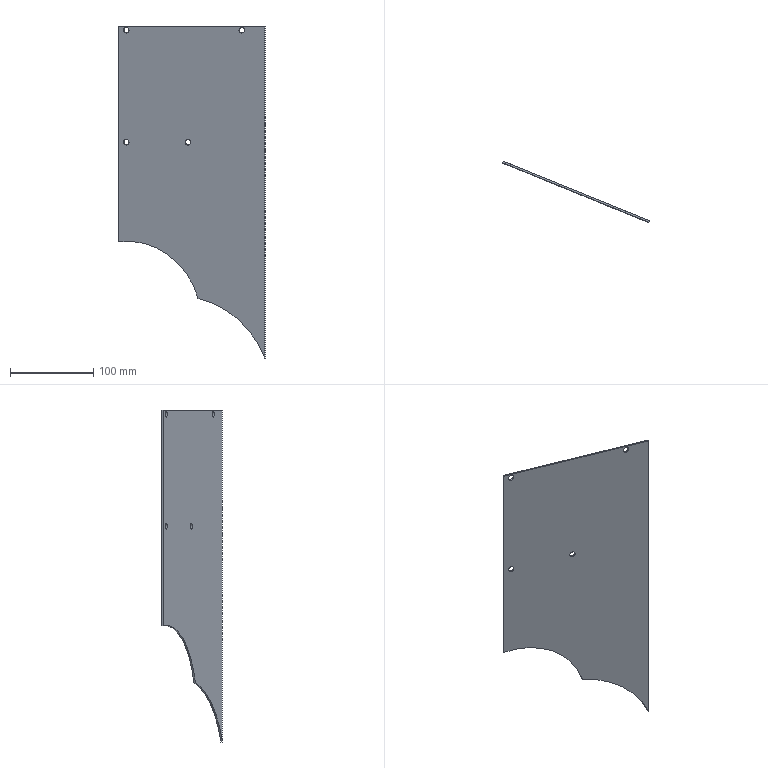Component | SolidWorks | InnerWing-1 | 1 solid | 15 faces | box 176.73 x 73.49 x 400 mm | volume 117704 mm3 | cylinder 10 | plane 5 | commonest cylinder face diameters 7 x8 244.108 x1 192.797 x1
build123d program:
from build123d import *

# Parameters (mm, degrees)
SKETCH1_W           = 190
SKETCH1_H           = 400
BOSS_EXTRUDE1_DEPTH = 2
SKETCH2_R           = 3.5
CUT_EXTRUDE1_DEPTH  = 2
CUT_EXTRUDE2_DEPTH  = 2


with BuildPart() as part:
    # Sketch1 → Boss-Extrude1 (new body)
    with BuildSketch(Plane.XY):
        with Locations((-110.229, 190)):
            Rectangle(SKETCH1_W, SKETCH1_H)
    extrude(amount=BOSS_EXTRUDE1_DEPTH)

    # Sketch2 → Cut-Extrude1 (cut)
    with BuildSketch(Plane.XY.offset(2)):
        with Locations((-195.229, -5)):
            Circle(SKETCH2_R)
        with Locations((-195.229, 130)):
            Circle(SKETCH2_R)
        with Locations((-115.229, 130)):
            Circle(SKETCH2_R)
        with Locations((-45.229, -5)):
            Circle(SKETCH2_R)
    extrude(amount=-CUT_EXTRUDE1_DEPTH, mode=Mode.SUBTRACT)

    # Sketch3 → Cut-Extrude2 (cut)
    with BuildSketch(Plane.XY.offset(2)):
        with BuildLine():
            Line((-205.229, 390), (-205.229, 250))
            ThreePointArc((-205.229, 250), (-141.251, 265.353), (-102.024, 318.174))
            ThreePointArc((-102.024, 318.174), (-49.844, 343.474), (-15.229, 390))
            Line((-15.229, 390), (-205.229, 390))
        make_face()
    extrude(amount=-CUT_EXTRUDE2_DEPTH, mode=Mode.SUBTRACT)


solid = part.part

# Placed as in the assembly
solid = solid.moved(Location((-18.038, -26.671, 107.182), (-90, 22.15, 0)))
STEP:
#1=COLOUR_RGB('',0.7922,0.8196,0.9333);
#2=FILL_AREA_STYLE_COLOUR('',#1);
#3=FILL_AREA_STYLE('',(#2));
#4=SURFACE_STYLE_FILL_AREA(#3);
#5=SURFACE_SIDE_STYLE('',(#4));
#6=SURFACE_STYLE_USAGE(.BOTH.,#5);
#7=PRESENTATION_STYLE_ASSIGNMENT((#6));
#8=CARTESIAN_POINT('',(-2.487,-0.3267,4.417));
#9=VERTEX_POINT('',#8);
#10=CARTESIAN_POINT('',(-2.232,-0.4306,4.417));
#11=VERTEX_POINT('',#10);
#12=CARTESIAN_POINT('',(-2.359,-0.3787,4.417));
#13=DIRECTION('',(0.377,0.9262,-0.));
#14=DIRECTION('',(0.9262,-0.377,0.));
#15=AXIS2_PLACEMENT_3D('',#12,#13,#14);
#16=CIRCLE('',#15,0.1378);
#17=EDGE_CURVE('',#9,#11,#16,.T.);
#18=ORIENTED_EDGE('',*,*,#17,.F.);
#19=CARTESIAN_POINT('',(-2.457,-0.2538,4.417));
#20=VERTEX_POINT('',#19);
#21=CARTESIAN_POINT('',(-2.487,-0.3267,4.417));
#22=DIRECTION('',(0.377,0.9262,-0.));
#23=VECTOR('',#22,39.37);
#24=LINE('',#21,#23);
#25=EDGE_CURVE('',#9,#20,#24,.T.);
#26=ORIENTED_EDGE('',*,*,#25,.T.);
#27=CARTESIAN_POINT('',(-2.202,-0.3577,4.417));
#28=VERTEX_POINT('',#27);
#29=CARTESIAN_POINT('',(-2.33,-0.3057,4.417));
#30=DIRECTION('',(0.377,0.9262,-0.));
#31=DIRECTION('',(0.9262,-0.377,0.));
#32=AXIS2_PLACEMENT_3D('',#29,#30,#31);
#33=CIRCLE('',#32,0.1378);
#34=EDGE_CURVE('',#20,#28,#33,.T.);
#35=ORIENTED_EDGE('',*,*,#34,.T.);
#36=CARTESIAN_POINT('',(-2.232,-0.4306,4.417));
#37=DIRECTION('',(0.377,0.9262,-0.));
#38=VECTOR('',#37,39.37);
#39=LINE('',#36,#38);
#40=EDGE_CURVE('',#11,#28,#39,.T.);
#41=ORIENTED_EDGE('',*,*,#40,.F.);
#42=EDGE_LOOP('',(#18,#26,#35,#41));
#43=FACE_OUTER_BOUND('',#42,.T.);
#44=CARTESIAN_POINT('',(-2.359,-0.3787,4.417));
#45=DIRECTION('',(0.377,0.9262,-0.));
#46=DIRECTION('',(0.9262,-0.377,0.));
#47=AXIS2_PLACEMENT_3D('',#44,#45,#46);
#48=CYLINDRICAL_SURFACE('',#47,0.1378);
#49=ADVANCED_FACE('',(#43),#48,.F.);
#50=CARTESIAN_POINT('',(-5.04,0.7124,-0.8983));
#51=VERTEX_POINT('',#50);
#52=CARTESIAN_POINT('',(-4.784,0.6084,-0.8983));
#53=VERTEX_POINT('',#52);
#54=CARTESIAN_POINT('',(-4.912,0.6604,-0.8983));
#55=DIRECTION('',(0.377,0.9262,-0.));
#56=DIRECTION('',(0.9262,-0.377,0.));
#57=AXIS2_PLACEMENT_3D('',#54,#55,#56);
#58=CIRCLE('',#57,0.1378);
#59=EDGE_CURVE('',#51,#53,#58,.T.);
#60=ORIENTED_EDGE('',*,*,#59,.F.);
#61=CARTESIAN_POINT('',(-5.01,0.7853,-0.8983));
#62=VERTEX_POINT('',#61);
#63=CARTESIAN_POINT('',(-5.04,0.7124,-0.8983));
#64=DIRECTION('',(0.377,0.9262,-0.));
#65=VECTOR('',#64,39.37);
#66=LINE('',#63,#65);
#67=EDGE_CURVE('',#51,#62,#66,.T.);
#68=ORIENTED_EDGE('',*,*,#67,.T.);
#69=CARTESIAN_POINT('',(-4.755,0.6814,-0.8983));
#70=VERTEX_POINT('',#69);
#71=CARTESIAN_POINT('',(-4.882,0.7333,-0.8983));
#72=DIRECTION('',(0.377,0.9262,-0.));
#73=DIRECTION('',(0.9262,-0.377,0.));
#74=AXIS2_PLACEMENT_3D('',#71,#72,#73);
#75=CIRCLE('',#74,0.1378);
#76=EDGE_CURVE('',#62,#70,#75,.T.);
#77=ORIENTED_EDGE('',*,*,#76,.T.);
#78=CARTESIAN_POINT('',(-4.784,0.6084,-0.8983));
#79=DIRECTION('',(0.377,0.9262,-0.));
#80=VECTOR('',#79,39.37);
#81=LINE('',#78,#80);
#82=EDGE_CURVE('',#53,#70,#81,.T.);
#83=ORIENTED_EDGE('',*,*,#82,.F.);
#84=EDGE_LOOP('',(#60,#68,#77,#83));
#85=FACE_OUTER_BOUND('',#84,.T.);
#86=CARTESIAN_POINT('',(-4.912,0.6604,-0.8983));
#87=DIRECTION('',(0.377,0.9262,-0.));
#88=DIRECTION('',(0.9262,-0.377,0.));
#89=AXIS2_PLACEMENT_3D('',#86,#87,#88);
#90=CYLINDRICAL_SURFACE('',#89,0.1378);
#91=ADVANCED_FACE('',(#85),#90,.F.);
#92=CARTESIAN_POINT('',(-7.957,1.9,-0.8983));
#93=VERTEX_POINT('',#92);
#94=CARTESIAN_POINT('',(-7.701,1.796,-0.8983));
#95=VERTEX_POINT('',#94);
#96=CARTESIAN_POINT('',(-7.829,1.848,-0.8983));
#97=DIRECTION('',(0.377,0.9262,-0.));
#98=DIRECTION('',(0.9262,-0.377,0.));
#99=AXIS2_PLACEMENT_3D('',#96,#97,#98);
#100=CIRCLE('',#99,0.1378);
#101=EDGE_CURVE('',#93,#95,#100,.T.);
#102=ORIENTED_EDGE('',*,*,#101,.F.);
#103=CARTESIAN_POINT('',(-7.927,1.973,-0.8983));
#104=VERTEX_POINT('',#103);
#105=CARTESIAN_POINT('',(-7.957,1.9,-0.8983));
#106=DIRECTION('',(0.377,0.9262,-0.));
#107=VECTOR('',#106,39.37);
#108=LINE('',#105,#107);
#109=EDGE_CURVE('',#93,#104,#108,.T.);
#110=ORIENTED_EDGE('',*,*,#109,.T.);
#111=CARTESIAN_POINT('',(-7.672,1.869,-0.8983));
#112=VERTEX_POINT('',#111);
#113=CARTESIAN_POINT('',(-7.799,1.921,-0.8983));
#114=DIRECTION('',(0.377,0.9262,-0.));
#115=DIRECTION('',(0.9262,-0.377,0.));
#116=AXIS2_PLACEMENT_3D('',#113,#114,#115);
#117=CIRCLE('',#116,0.1378);
#118=EDGE_CURVE('',#104,#112,#117,.T.);
#119=ORIENTED_EDGE('',*,*,#118,.T.);
#120=CARTESIAN_POINT('',(-7.701,1.796,-0.8983));
#121=DIRECTION('',(0.377,0.9262,-0.));
#122=VECTOR('',#121,39.37);
#123=LINE('',#120,#122);
#124=EDGE_CURVE('',#95,#112,#123,.T.);
#125=ORIENTED_EDGE('',*,*,#124,.F.);
#126=EDGE_LOOP('',(#102,#110,#119,#125));
#127=FACE_OUTER_BOUND('',#126,.T.);
#128=CARTESIAN_POINT('',(-7.829,1.848,-0.8983));
#129=DIRECTION('',(0.377,0.9262,-0.));
#130=DIRECTION('',(0.9262,-0.377,0.));
#131=AXIS2_PLACEMENT_3D('',#128,#129,#130);
#132=CYLINDRICAL_SURFACE('',#131,0.1378);
#133=ADVANCED_FACE('',(#127),#132,.F.);
#134=CARTESIAN_POINT('',(-7.957,1.9,4.417));
#135=VERTEX_POINT('',#134);
#136=CARTESIAN_POINT('',(-7.701,1.796,4.417));
#137=VERTEX_POINT('',#136);
#138=CARTESIAN_POINT('',(-7.829,1.848,4.417));
#139=DIRECTION('',(0.377,0.9262,-0.));
#140=DIRECTION('',(0.9262,-0.377,0.));
#141=AXIS2_PLACEMENT_3D('',#138,#139,#140);
#142=CIRCLE('',#141,0.1378);
#143=EDGE_CURVE('',#135,#137,#142,.T.);
#144=ORIENTED_EDGE('',*,*,#143,.F.);
#145=CARTESIAN_POINT('',(-7.927,1.973,4.417));
#146=VERTEX_POINT('',#145);
#147=CARTESIAN_POINT('',(-7.957,1.9,4.417));
#148=DIRECTION('',(0.377,0.9262,-0.));
#149=VECTOR('',#148,39.37);
#150=LINE('',#147,#149);
#151=EDGE_CURVE('',#135,#146,#150,.T.);
#152=ORIENTED_EDGE('',*,*,#151,.T.);
#153=CARTESIAN_POINT('',(-7.672,1.869,4.417));
#154=VERTEX_POINT('',#153);
#155=CARTESIAN_POINT('',(-7.799,1.921,4.417));
#156=DIRECTION('',(0.377,0.9262,-0.));
#157=DIRECTION('',(0.9262,-0.377,0.));
#158=AXIS2_PLACEMENT_3D('',#155,#156,#157);
#159=CIRCLE('',#158,0.1378);
#160=EDGE_CURVE('',#146,#154,#159,.T.);
#161=ORIENTED_EDGE('',*,*,#160,.T.);
#162=CARTESIAN_POINT('',(-7.701,1.796,4.417));
#163=DIRECTION('',(0.377,0.9262,-0.));
#164=VECTOR('',#163,39.37);
#165=LINE('',#162,#164);
#166=EDGE_CURVE('',#137,#154,#165,.T.);
#167=ORIENTED_EDGE('',*,*,#166,.F.);
#168=EDGE_LOOP('',(#144,#152,#161,#167));
#169=FACE_OUTER_BOUND('',#168,.T.);
#170=CARTESIAN_POINT('',(-7.829,1.848,4.417));
#171=DIRECTION('',(0.377,0.9262,-0.));
#172=DIRECTION('',(0.9262,-0.377,0.));
#173=AXIS2_PLACEMENT_3D('',#170,#171,#172);
#174=CYLINDRICAL_SURFACE('',#173,0.1378);
#175=ADVANCED_FACE('',(#169),#174,.F.);
#176=CARTESIAN_POINT('',(-8.164,2.069,-5.623));
#177=VERTEX_POINT('',#176);
#178=CARTESIAN_POINT('',(-8.164,2.069,4.613));
#179=VERTEX_POINT('',#178);
#180=CARTESIAN_POINT('',(-8.164,2.069,4.613));
#181=DIRECTION('',(-0.,0.,1.));
#182=VECTOR('',#181,39.37);
#183=LINE('',#180,#182);
#184=EDGE_CURVE('',#177,#179,#183,.T.);
#185=ORIENTED_EDGE('',*,*,#184,.F.);
#186=CARTESIAN_POINT('',(-8.194,1.996,-5.623));
#187=VERTEX_POINT('',#186);
#188=CARTESIAN_POINT('',(-8.194,1.996,-5.623));
#189=DIRECTION('',(0.377,0.9262,-0.));
#190=VECTOR('',#189,39.37);
#191=LINE('',#188,#190);
#192=EDGE_CURVE('',#187,#177,#191,.T.);
#193=ORIENTED_EDGE('',*,*,#192,.F.);
#194=CARTESIAN_POINT('',(-8.194,1.996,4.613));
#195=VERTEX_POINT('',#194);
#196=CARTESIAN_POINT('',(-8.194,1.996,4.613));
#197=DIRECTION('',(-0.,0.,1.));
#198=VECTOR('',#197,39.37);
#199=LINE('',#196,#198);
#200=EDGE_CURVE('',#187,#195,#199,.T.);
#201=ORIENTED_EDGE('',*,*,#200,.T.);
#202=CARTESIAN_POINT('',(-8.164,2.069,4.613));
#203=DIRECTION('',(-0.377,-0.9262,0.));
#204=VECTOR('',#203,39.37);
#205=LINE('',#202,#204);
#206=EDGE_CURVE('',#179,#195,#205,.T.);
#207=ORIENTED_EDGE('',*,*,#206,.F.);
#208=EDGE_LOOP('',(#185,#193,#201,#207));
#209=FACE_OUTER_BOUND('',#208,.T.);
#210=CARTESIAN_POINT('',(-8.164,2.069,4.613));
#211=DIRECTION('',(0.9262,-0.377,0.));
#212=DIRECTION('',(-0.377,-0.9262,0.));
#213=AXIS2_PLACEMENT_3D('',#210,#211,#212);
#214=PLANE('',#213);
#215=ADVANCED_FACE('',(#209),#214,.F.);
#216=CARTESIAN_POINT('',(-1.265,-0.824,4.613));
#217=VERTEX_POINT('',#216);
#218=CARTESIAN_POINT('',(-8.194,1.996,4.613));
#219=DIRECTION('',(0.9262,-0.377,0.));
#220=VECTOR('',#219,39.37);
#221=LINE('',#218,#220);
#222=EDGE_CURVE('',#195,#217,#221,.T.);
#223=ORIENTED_EDGE('',*,*,#222,.T.);
#224=CARTESIAN_POINT('',(-1.236,-0.7511,4.613));
#225=VERTEX_POINT('',#224);
#226=CARTESIAN_POINT('',(-1.236,-0.7511,4.613));
#227=DIRECTION('',(-0.377,-0.9262,0.));
#228=VECTOR('',#227,39.37);
#229=LINE('',#226,#228);
#230=EDGE_CURVE('',#225,#217,#229,.T.);
#231=ORIENTED_EDGE('',*,*,#230,.F.);
#232=CARTESIAN_POINT('',(-8.164,2.069,4.613));
#233=DIRECTION('',(0.9262,-0.377,0.));
#234=VECTOR('',#233,39.37);
#235=LINE('',#232,#234);
#236=EDGE_CURVE('',#179,#225,#235,.T.);
#237=ORIENTED_EDGE('',*,*,#236,.F.);
#238=ORIENTED_EDGE('',*,*,#206,.T.);
#239=EDGE_LOOP('',(#223,#231,#237,#238));
#240=FACE_OUTER_BOUND('',#239,.T.);
#241=CARTESIAN_POINT('',(-8.164,2.069,4.613));
#242=DIRECTION('',(0.,-0.,-1.));
#243=DIRECTION('',(-0.9262,0.377,-0.));
#244=AXIS2_PLACEMENT_3D('',#241,#242,#243);
#245=PLANE('',#244);
#246=ADVANCED_FACE('',(#240),#245,.F.);
#247=CARTESIAN_POINT('',(-1.265,-0.824,-11.135));
#248=VERTEX_POINT('',#247);
#249=CARTESIAN_POINT('',(-1.265,-0.824,4.613));
#250=DIRECTION('',(0.,-0.,-1.));
#251=VECTOR('',#250,39.37);
#252=LINE('',#249,#251);
#253=EDGE_CURVE('',#217,#248,#252,.T.);
#254=ORIENTED_EDGE('',*,*,#253,.T.);
#255=CARTESIAN_POINT('',(-1.236,-0.7511,-11.135));
#256=VERTEX_POINT('',#255);
#257=CARTESIAN_POINT('',(-1.236,-0.7511,-11.135));
#258=DIRECTION('',(-0.377,-0.9262,0.));
#259=VECTOR('',#258,39.37);
#260=LINE('',#257,#259);
#261=EDGE_CURVE('',#256,#248,#260,.T.);
#262=ORIENTED_EDGE('',*,*,#261,.F.);
#263=CARTESIAN_POINT('',(-1.236,-0.7511,4.613));
#264=DIRECTION('',(0.,-0.,-1.));
#265=VECTOR('',#264,39.37);
#266=LINE('',#263,#265);
#267=EDGE_CURVE('',#225,#256,#266,.T.);
#268=ORIENTED_EDGE('',*,*,#267,.F.);
#269=ORIENTED_EDGE('',*,*,#230,.T.);
#270=EDGE_LOOP('',(#254,#262,#268,#269));
#271=FACE_OUTER_BOUND('',#270,.T.);
#272=CARTESIAN_POINT('',(-1.236,-0.7511,4.613));
#273=DIRECTION('',(-0.9262,0.377,-0.));
#274=DIRECTION('',(0.377,0.9262,-0.));
#275=AXIS2_PLACEMENT_3D('',#272,#273,#274);
#276=PLANE('',#275);
#277=ADVANCED_FACE('',(#271),#276,.F.);
#278=CARTESIAN_POINT('',(-2.33,-0.3057,4.417));
#279=DIRECTION('',(0.377,0.9262,-0.));
#280=DIRECTION('',(0.9262,-0.377,0.));
#281=AXIS2_PLACEMENT_3D('',#278,#279,#280);
#282=CIRCLE('',#281,0.1378);
#283=EDGE_CURVE('',#28,#20,#282,.T.);
#284=ORIENTED_EDGE('',*,*,#283,.F.);
#285=ORIENTED_EDGE('',*,*,#34,.F.);
#286=EDGE_LOOP('',(#284,#285));
#287=FACE_BOUND('',#286,.T.);
#288=CARTESIAN_POINT('',(-4.882,0.7333,-0.8983));
#289=DIRECTION('',(0.377,0.9262,-0.));
#290=DIRECTION('',(0.9262,-0.377,0.));
#291=AXIS2_PLACEMENT_3D('',#288,#289,#290);
#292=CIRCLE('',#291,0.1378);
#293=EDGE_CURVE('',#70,#62,#292,.T.);
#294=ORIENTED_EDGE('',*,*,#293,.F.);
#295=ORIENTED_EDGE('',*,*,#76,.F.);
#296=EDGE_LOOP('',(#294,#295));
#297=FACE_BOUND('',#296,.T.);
#298=CARTESIAN_POINT('',(-7.799,1.921,-0.8983));
#299=DIRECTION('',(0.377,0.9262,-0.));
#300=DIRECTION('',(0.9262,-0.377,0.));
#301=AXIS2_PLACEMENT_3D('',#298,#299,#300);
#302=CIRCLE('',#301,0.1378);
#303=EDGE_CURVE('',#112,#104,#302,.T.);
#304=ORIENTED_EDGE('',*,*,#303,.F.);
#305=ORIENTED_EDGE('',*,*,#118,.F.);
#306=EDGE_LOOP('',(#304,#305));
#307=FACE_BOUND('',#306,.T.);
#308=CARTESIAN_POINT('',(-7.799,1.921,4.417));
#309=DIRECTION('',(0.377,0.9262,-0.));
#310=DIRECTION('',(0.9262,-0.377,0.));
#311=AXIS2_PLACEMENT_3D('',#308,#309,#310);
#312=CIRCLE('',#311,0.1378);
#313=EDGE_CURVE('',#154,#146,#312,.T.);
#314=ORIENTED_EDGE('',*,*,#313,.F.);
#315=ORIENTED_EDGE('',*,*,#160,.F.);
#316=EDGE_LOOP('',(#314,#315));
#317=FACE_BOUND('',#316,.T.);
#318=ORIENTED_EDGE('',*,*,#267,.T.);
#319=CARTESIAN_POINT('',(-4.401,0.5373,-8.307));
#320=VERTEX_POINT('',#319);
#321=CARTESIAN_POINT('',(-5.335,0.9178,-13.005));
#322=DIRECTION('',(0.377,0.9262,-0.));
#323=DIRECTION('',(0.9262,-0.377,0.));
#324=AXIS2_PLACEMENT_3D('',#321,#322,#323);
#325=CIRCLE('',#324,4.805);
#326=EDGE_CURVE('',#320,#256,#325,.T.);
#327=ORIENTED_EDGE('',*,*,#326,.F.);
#328=CARTESIAN_POINT('',(-7.769,1.908,-9.394));
#329=DIRECTION('',(0.377,0.9262,-0.));
#330=DIRECTION('',(0.9262,-0.377,0.));
#331=AXIS2_PLACEMENT_3D('',#328,#329,#330);
#332=CIRCLE('',#331,3.795);
#333=EDGE_CURVE('',#177,#320,#332,.T.);
#334=ORIENTED_EDGE('',*,*,#333,.F.);
#335=ORIENTED_EDGE('',*,*,#184,.T.);
#336=ORIENTED_EDGE('',*,*,#236,.T.);
#337=EDGE_LOOP('',(#318,#327,#334,#335,#336));
#338=FACE_OUTER_BOUND('',#337,.T.);
#339=CARTESIAN_POINT('',(-0.6805,-0.9771,4.22));
#340=DIRECTION('',(-0.377,-0.9262,0.));
#341=DIRECTION('',(-0.9262,0.377,-0.));
#342=AXIS2_PLACEMENT_3D('',#339,#340,#341);
#343=PLANE('',#342);
#344=ADVANCED_FACE('',(#287,#297,#307,#317,#338),#343,.F.);
#345=CARTESIAN_POINT('',(-4.43,0.4644,-8.307));
#346=VERTEX_POINT('',#345);
#347=CARTESIAN_POINT('',(-5.365,0.8449,-13.005));
#348=DIRECTION('',(0.377,0.9262,-0.));
#349=DIRECTION('',(0.9262,-0.377,0.));
#350=AXIS2_PLACEMENT_3D('',#347,#348,#349);
#351=CIRCLE('',#350,4.805);
#352=EDGE_CURVE('',#346,#248,#351,.T.);
#353=ORIENTED_EDGE('',*,*,#352,.T.);
#354=ORIENTED_EDGE('',*,*,#253,.F.);
#355=ORIENTED_EDGE('',*,*,#222,.F.);
#356=ORIENTED_EDGE('',*,*,#200,.F.);
#357=CARTESIAN_POINT('',(-7.798,1.835,-9.394));
#358=DIRECTION('',(0.377,0.9262,-0.));
#359=DIRECTION('',(0.9262,-0.377,0.));
#360=AXIS2_PLACEMENT_3D('',#357,#358,#359);
#361=CIRCLE('',#360,3.795);
#362=EDGE_CURVE('',#187,#346,#361,.T.);
#363=ORIENTED_EDGE('',*,*,#362,.T.);
#364=EDGE_LOOP('',(#353,#354,#355,#356,#363));
#365=FACE_OUTER_BOUND('',#364,.T.);
#366=CARTESIAN_POINT('',(-2.359,-0.3787,4.417));
#367=DIRECTION('',(0.377,0.9262,-0.));
#368=DIRECTION('',(0.9262,-0.377,0.));
#369=AXIS2_PLACEMENT_3D('',#366,#367,#368);
#370=CIRCLE('',#369,0.1378);
#371=EDGE_CURVE('',#11,#9,#370,.T.);
#372=ORIENTED_EDGE('',*,*,#371,.T.);
#373=ORIENTED_EDGE('',*,*,#17,.T.);
#374=EDGE_LOOP('',(#372,#373));
#375=FACE_BOUND('',#374,.T.);
#376=CARTESIAN_POINT('',(-4.912,0.6604,-0.8983));
#377=DIRECTION('',(0.377,0.9262,-0.));
#378=DIRECTION('',(0.9262,-0.377,0.));
#379=AXIS2_PLACEMENT_3D('',#376,#377,#378);
#380=CIRCLE('',#379,0.1378);
#381=EDGE_CURVE('',#53,#51,#380,.T.);
#382=ORIENTED_EDGE('',*,*,#381,.T.);
#383=ORIENTED_EDGE('',*,*,#59,.T.);
#384=EDGE_LOOP('',(#382,#383));
#385=FACE_BOUND('',#384,.T.);
#386=CARTESIAN_POINT('',(-7.829,1.848,-0.8983));
#387=DIRECTION('',(0.377,0.9262,-0.));
#388=DIRECTION('',(0.9262,-0.377,0.));
#389=AXIS2_PLACEMENT_3D('',#386,#387,#388);
#390=CIRCLE('',#389,0.1378);
#391=EDGE_CURVE('',#95,#93,#390,.T.);
#392=ORIENTED_EDGE('',*,*,#391,.T.);
#393=ORIENTED_EDGE('',*,*,#101,.T.);
#394=EDGE_LOOP('',(#392,#393));
#395=FACE_BOUND('',#394,.T.);
#396=CARTESIAN_POINT('',(-7.829,1.848,4.417));
#397=DIRECTION('',(0.377,0.9262,-0.));
#398=DIRECTION('',(0.9262,-0.377,0.));
#399=AXIS2_PLACEMENT_3D('',#396,#397,#398);
#400=CIRCLE('',#399,0.1378);
#401=EDGE_CURVE('',#137,#135,#400,.T.);
#402=ORIENTED_EDGE('',*,*,#401,.T.);
#403=ORIENTED_EDGE('',*,*,#143,.T.);
#404=EDGE_LOOP('',(#402,#403));
#405=FACE_BOUND('',#404,.T.);
#406=CARTESIAN_POINT('',(-0.7102,-1.05,4.22));
#407=DIRECTION('',(-0.377,-0.9262,0.));
#408=DIRECTION('',(-0.9262,0.377,-0.));
#409=AXIS2_PLACEMENT_3D('',#406,#407,#408);
#410=PLANE('',#409);
#411=ADVANCED_FACE('',(#365,#375,#385,#395,#405),#410,.T.);
#412=ORIENTED_EDGE('',*,*,#151,.F.);
#413=ORIENTED_EDGE('',*,*,#401,.F.);
#414=ORIENTED_EDGE('',*,*,#166,.T.);
#415=ORIENTED_EDGE('',*,*,#313,.T.);
#416=EDGE_LOOP('',(#412,#413,#414,#415));
#417=FACE_OUTER_BOUND('',#416,.T.);
#418=CARTESIAN_POINT('',(-7.829,1.848,4.417));
#419=DIRECTION('',(0.377,0.9262,-0.));
#420=DIRECTION('',(0.9262,-0.377,0.));
#421=AXIS2_PLACEMENT_3D('',#418,#419,#420);
#422=CYLINDRICAL_SURFACE('',#421,0.1378);
#423=ADVANCED_FACE('',(#417),#422,.F.);
#424=ORIENTED_EDGE('',*,*,#109,.F.);
#425=ORIENTED_EDGE('',*,*,#391,.F.);
#426=ORIENTED_EDGE('',*,*,#124,.T.);
#427=ORIENTED_EDGE('',*,*,#303,.T.);
#428=EDGE_LOOP('',(#424,#425,#426,#427));
#429=FACE_OUTER_BOUND('',#428,.T.);
#430=CARTESIAN_POINT('',(-7.829,1.848,-0.8983));
#431=DIRECTION('',(0.377,0.9262,-0.));
#432=DIRECTION('',(0.9262,-0.377,0.));
#433=AXIS2_PLACEMENT_3D('',#430,#431,#432);
#434=CYLINDRICAL_SURFACE('',#433,0.1378);
#435=ADVANCED_FACE('',(#429),#434,.F.);
#436=ORIENTED_EDGE('',*,*,#67,.F.);
#437=ORIENTED_EDGE('',*,*,#381,.F.);
#438=ORIENTED_EDGE('',*,*,#82,.T.);
#439=ORIENTED_EDGE('',*,*,#293,.T.);
#440=EDGE_LOOP('',(#436,#437,#438,#439));
#441=FACE_OUTER_BOUND('',#440,.T.);
#442=CARTESIAN_POINT('',(-4.912,0.6604,-0.8983));
#443=DIRECTION('',(0.377,0.9262,-0.));
#444=DIRECTION('',(0.9262,-0.377,0.));
#445=AXIS2_PLACEMENT_3D('',#442,#443,#444);
#446=CYLINDRICAL_SURFACE('',#445,0.1378);
#447=ADVANCED_FACE('',(#441),#446,.F.);
#448=ORIENTED_EDGE('',*,*,#25,.F.);
#449=ORIENTED_EDGE('',*,*,#371,.F.);
#450=ORIENTED_EDGE('',*,*,#40,.T.);
#451=ORIENTED_EDGE('',*,*,#283,.T.);
#452=EDGE_LOOP('',(#448,#449,#450,#451));
#453=FACE_OUTER_BOUND('',#452,.T.);
#454=CARTESIAN_POINT('',(-2.359,-0.3787,4.417));
#455=DIRECTION('',(0.377,0.9262,-0.));
#456=DIRECTION('',(0.9262,-0.377,0.));
#457=AXIS2_PLACEMENT_3D('',#454,#455,#456);
#458=CYLINDRICAL_SURFACE('',#457,0.1378);
#459=ADVANCED_FACE('',(#453),#458,.F.);
#460=ORIENTED_EDGE('',*,*,#326,.T.);
#461=ORIENTED_EDGE('',*,*,#261,.T.);
#462=ORIENTED_EDGE('',*,*,#352,.F.);
#463=CARTESIAN_POINT('',(-4.43,0.4644,-8.307));
#464=DIRECTION('',(0.377,0.9262,-0.));
#465=VECTOR('',#464,39.37);
#466=LINE('',#463,#465);
#467=EDGE_CURVE('',#346,#320,#466,.T.);
#468=ORIENTED_EDGE('',*,*,#467,.T.);
#469=EDGE_LOOP('',(#460,#461,#462,#468));
#470=FACE_OUTER_BOUND('',#469,.T.);
#471=CARTESIAN_POINT('',(-5.365,0.8449,-13.005));
#472=DIRECTION('',(0.377,0.9262,-0.));
#473=DIRECTION('',(0.9262,-0.377,0.));
#474=AXIS2_PLACEMENT_3D('',#471,#472,#473);
#475=CYLINDRICAL_SURFACE('',#474,4.805);
#476=ADVANCED_FACE('',(#470),#475,.F.);
#477=ORIENTED_EDGE('',*,*,#333,.T.);
#478=ORIENTED_EDGE('',*,*,#467,.F.);
#479=ORIENTED_EDGE('',*,*,#362,.F.);
#480=ORIENTED_EDGE('',*,*,#192,.T.);
#481=EDGE_LOOP('',(#477,#478,#479,#480));
#482=FACE_OUTER_BOUND('',#481,.T.);
#483=CARTESIAN_POINT('',(-7.798,1.835,-9.394));
#484=DIRECTION('',(0.377,0.9262,-0.));
#485=DIRECTION('',(0.9262,-0.377,0.));
#486=AXIS2_PLACEMENT_3D('',#483,#484,#485);
#487=CYLINDRICAL_SURFACE('',#486,3.795);
#488=ADVANCED_FACE('',(#482),#487,.F.);
#489=CLOSED_SHELL('',(#49,#91,#133,#175,#215,#246,#277,#344,#411,#423,#435,#447,#459,#476,#488));
#490=MANIFOLD_SOLID_BREP('',#489);
#491=STYLED_ITEM('',(#7),#490);
#492=PRESENTATION_LAYER_ASSIGNMENT('','',(#491));
#493=(LENGTH_UNIT()NAMED_UNIT(*)SI_UNIT($,.METRE.));
#494=LENGTH_MEASURE_WITH_UNIT(LENGTH_MEASURE(0.0254),#493);
#495=DIMENSIONAL_EXPONENTS(1.,0.,0.,0.,0.,0.,0.);
#496=(CONVERSION_BASED_UNIT('',#494)LENGTH_UNIT()NAMED_UNIT(#495));
#497=UNCERTAINTY_MEASURE_WITH_UNIT(LENGTH_MEASURE(0.00001),#496,'','');
#498=(NAMED_UNIT(*)PLANE_ANGLE_UNIT()SI_UNIT($,.RADIAN.));
#499=(NAMED_UNIT(*)SI_UNIT($,.STERADIAN.)SOLID_ANGLE_UNIT());
#500=(GEOMETRIC_REPRESENTATION_CONTEXT(3)GLOBAL_UNCERTAINTY_ASSIGNED_CONTEXT((#497))GLOBAL_UNIT_ASSIGNED_CONTEXT((#496,#498,#499))REPRESENTATION_CONTEXT('',''));
#501=MECHANICAL_DESIGN_GEOMETRIC_PRESENTATION_REPRESENTATION('',(#491),#500);
#502=CARTESIAN_POINT('',(0.,0.,0.));
#503=DIRECTION('',(0.,0.,1.));
#504=DIRECTION('',(1.,0.,0.));
#505=AXIS2_PLACEMENT_3D('',#502,#503,#504);
#506=(LENGTH_UNIT()NAMED_UNIT(*)SI_UNIT($,.METRE.));
#507=LENGTH_MEASURE_WITH_UNIT(LENGTH_MEASURE(0.0254),#506);
#508=DIMENSIONAL_EXPONENTS(1.,0.,0.,0.,0.,0.,0.);
#509=(CONVERSION_BASED_UNIT('',#507)LENGTH_UNIT()NAMED_UNIT(#508));
#510=UNCERTAINTY_MEASURE_WITH_UNIT(LENGTH_MEASURE(0.00001),#509,'','');
#511=(NAMED_UNIT(*)PLANE_ANGLE_UNIT()SI_UNIT($,.RADIAN.));
#512=(NAMED_UNIT(*)SI_UNIT($,.STERADIAN.)SOLID_ANGLE_UNIT());
#513=(GEOMETRIC_REPRESENTATION_CONTEXT(3)GLOBAL_UNCERTAINTY_ASSIGNED_CONTEXT((#510))GLOBAL_UNIT_ASSIGNED_CONTEXT((#509,#511,#512))REPRESENTATION_CONTEXT('',''));
#514=ADVANCED_BREP_SHAPE_REPRESENTATION('',(#490,#505),#513);